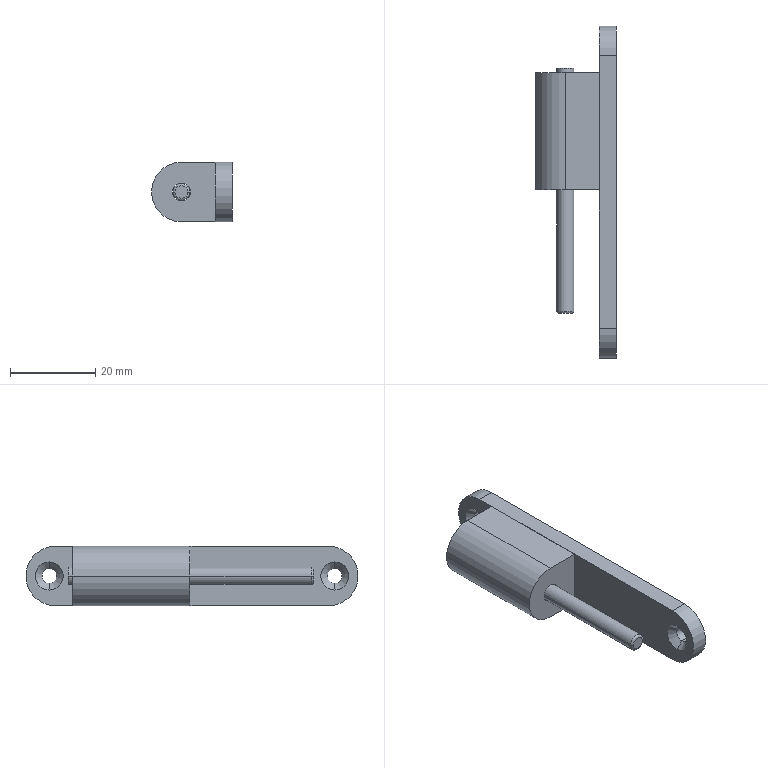Component | SolidWorks | MGL-PACK-03-00Fixture-1_MGL-PACK-03-07Hinge-1_MGL-PACK-03-07-01HingePart1-1 | 3 solids | 29 faces | box 19 x 78 x 14 mm | volume 9629 mm3 | cylinder 12 | plane 11 | cone 4 | torus 2 | commonest cylinder face diameters 14 x4 3.4 x4 4 x2 4.2 x2
build123d program:
from build123d import *

# Parameters (mm, degrees)
BOSS_EXTRUDE1_DEPTH                          = 4
BOSS_EXTRUDE2_DEPTH                          = 27.5
SKETCH5_R                                    = 2.1
CUT_EXTRUDE1_DEPTH                           = 27.5
SKETCH6_R                                    = 2
BOSS_EXTRUDE3_DEPTH                          = 57.5
FILLET1_R                                    = 0.5
HOLE_SIZE_ACCORDING_TO_PHILLIPS_COUN_2_COUNT = 2
HOLE_SIZE_ACCORDING_TO_PHILLIPS_COUN_2_PITCH = 67


with BuildPart() as part:
    # Sketch1 → Boss-Extrude1 (new body)
    with BuildSketch(Plane.XY):
        with BuildLine():
            Line((-7, 32), (-7, -32))
            ThreePointArc((-7, -32), (0, -39), (7, -32))
            Line((7, -32), (7, 32))
            ThreePointArc((7, 32), (0, 39), (-7, 32))
        make_face()
    extrude(amount=BOSS_EXTRUDE1_DEPTH)

    # Sketch7 → Hole Size according to Phillips counters (revolve, cut)
    with BuildSketch(Plane(origin=(0, 33.5, 4), x_dir=(0, -1, 0), z_dir=(1, 0, 0))):
        Polygon((0, 0), (0, 4), (1.7, 4), (1.7, 1.6), (3.3, 0), align=None)
    hole_size_according_to_phillips_counters = revolve(axis=Axis((0, 33.5, 10.35), (0, 0, -1)), mode=Mode.SUBTRACT)

    # Hole Size according to Phillips coun 2: Hole Size according to Phillips counters ×2
    with Locations(*[(0, -i * HOLE_SIZE_ACCORDING_TO_PHILLIPS_COUN_2_PITCH, 0) for i in range(1, HOLE_SIZE_ACCORDING_TO_PHILLIPS_COUN_2_COUNT)]):
        add(hole_size_according_to_phillips_counters, mode=Mode.SUBTRACT)


with BuildPart() as body_2:
    # Sketch2 → Boss-Extrude2 (new body)
    with BuildSketch(Plane(origin=(0, 28, 0), x_dir=(1, 0, 0), z_dir=(0, 1, 0))):
        with BuildLine():
            Line((-7, -4), (7, -4))
            Line((7, -4), (7, -12))
            ThreePointArc((7, -12), (0, -19), (-7, -12))
            Line((-7, -12), (-7, -4))
        make_face()
    extrude(amount=-BOSS_EXTRUDE2_DEPTH)

    # Sketch5 → Cut-Extrude1 (cut)
    with BuildSketch(Plane(origin=(0, 28, 0), x_dir=(1, 0, 0), z_dir=(0, 1, 0))):
        with Locations(Location((0, -12, 0), (0, 0, 270))):
            Circle(SKETCH5_R)
    extrude(amount=-CUT_EXTRUDE1_DEPTH, mode=Mode.SUBTRACT)


with BuildPart() as body_3:
    # Sketch6 → Boss-Extrude3 (new body)
    with BuildSketch(Plane(origin=(0, 29, 0), x_dir=(1, 0, 0), z_dir=(0, 1, 0))):
        with Locations(Location((0, -12, 0), (0, 0, 270))):
            Circle(SKETCH6_R)
    extrude(amount=-BOSS_EXTRUDE3_DEPTH)

    # Fillet1
    fillet1_edges = [body_3.edges().sort_by_distance(p)[0] for p in [
        (0, -28.5, 10),
    ]]
    fillet(fillet1_edges, radius=FILLET1_R)


solid = Compound([part.part, body_2.part, body_3.part])

# Placed as in the assembly
solid = solid.moved(Location((279.5, 0, 1.7), (0, -90, 0)))
STEP:
#1=COLOUR_RGB('',0.7922,0.8196,0.9333);
#2=FILL_AREA_STYLE_COLOUR('',#1);
#3=FILL_AREA_STYLE('',(#2));
#4=SURFACE_STYLE_FILL_AREA(#3);
#5=SURFACE_SIDE_STYLE('',(#4));
#6=SURFACE_STYLE_USAGE(.BOTH.,#5);
#7=PRESENTATION_STYLE_ASSIGNMENT((#6));
#8=CARTESIAN_POINT('',(10.909,1.319,0.));
#9=VERTEX_POINT('',#8);
#10=CARTESIAN_POINT('',(10.909,1.319,0.1339));
#11=VERTEX_POINT('',#10);
#12=CARTESIAN_POINT('',(10.909,1.319,0.06693));
#13=DIRECTION('',(-1.,-0.,0.));
#14=DIRECTION('',(0.,0.,1.));
#15=AXIS2_PLACEMENT_3D('',#12,#13,#14);
#16=CIRCLE('',#15,0.06693);
#17=EDGE_CURVE('',#9,#11,#16,.T.);
#18=ORIENTED_EDGE('',*,*,#17,.F.);
#19=CARTESIAN_POINT('',(10.846,1.319,-0.06299));
#20=VERTEX_POINT('',#19);
#21=CARTESIAN_POINT('',(10.846,1.319,-0.06299));
#22=DIRECTION('',(-0.7071,-0.,-0.7071));
#23=VECTOR('',#22,39.37);
#24=LINE('',#21,#23);
#25=EDGE_CURVE('',#9,#20,#24,.T.);
#26=ORIENTED_EDGE('',*,*,#25,.T.);
#27=CARTESIAN_POINT('',(10.846,1.319,0.1969));
#28=VERTEX_POINT('',#27);
#29=CARTESIAN_POINT('',(10.846,1.319,0.06693));
#30=DIRECTION('',(-1.,-0.,0.));
#31=DIRECTION('',(0.,0.,1.));
#32=AXIS2_PLACEMENT_3D('',#29,#30,#31);
#33=CIRCLE('',#32,0.1299);
#34=EDGE_CURVE('',#20,#28,#33,.T.);
#35=ORIENTED_EDGE('',*,*,#34,.T.);
#36=CARTESIAN_POINT('',(10.846,1.319,0.1969));
#37=DIRECTION('',(-0.7071,-0.,0.7071));
#38=VECTOR('',#37,39.37);
#39=LINE('',#36,#38);
#40=EDGE_CURVE('',#11,#28,#39,.T.);
#41=ORIENTED_EDGE('',*,*,#40,.F.);
#42=EDGE_LOOP('',(#18,#26,#35,#41));
#43=FACE_OUTER_BOUND('',#42,.T.);
#44=CARTESIAN_POINT('',(10.846,1.319,0.06693));
#45=DIRECTION('',(-1.,-0.,0.));
#46=DIRECTION('',(0.,0.,1.));
#47=AXIS2_PLACEMENT_3D('',#44,#45,#46);
#48=CONICAL_SURFACE('',#47,0.1299,0.7854);
#49=ADVANCED_FACE('',(#43),#48,.F.);
#50=CARTESIAN_POINT('',(11.004,1.319,0.));
#51=VERTEX_POINT('',#50);
#52=CARTESIAN_POINT('',(11.004,1.319,0.1339));
#53=VERTEX_POINT('',#52);
#54=CARTESIAN_POINT('',(11.004,1.319,0.06693));
#55=DIRECTION('',(-1.,-0.,0.));
#56=DIRECTION('',(0.,0.,1.));
#57=AXIS2_PLACEMENT_3D('',#54,#55,#56);
#58=CIRCLE('',#57,0.06693);
#59=EDGE_CURVE('',#51,#53,#58,.T.);
#60=ORIENTED_EDGE('',*,*,#59,.F.);
#61=CARTESIAN_POINT('',(10.846,1.319,0.));
#62=DIRECTION('',(-1.,-0.,0.));
#63=VECTOR('',#62,39.37);
#64=LINE('',#61,#63);
#65=EDGE_CURVE('',#51,#9,#64,.T.);
#66=ORIENTED_EDGE('',*,*,#65,.T.);
#67=ORIENTED_EDGE('',*,*,#17,.T.);
#68=CARTESIAN_POINT('',(10.846,1.319,0.1339));
#69=DIRECTION('',(-1.,-0.,0.));
#70=VECTOR('',#69,39.37);
#71=LINE('',#68,#70);
#72=EDGE_CURVE('',#53,#11,#71,.T.);
#73=ORIENTED_EDGE('',*,*,#72,.F.);
#74=EDGE_LOOP('',(#60,#66,#67,#73));
#75=FACE_OUTER_BOUND('',#74,.T.);
#76=CARTESIAN_POINT('',(10.846,1.319,0.06693));
#77=DIRECTION('',(-1.,-0.,0.));
#78=DIRECTION('',(0.,0.,1.));
#79=AXIS2_PLACEMENT_3D('',#76,#77,#78);
#80=CYLINDRICAL_SURFACE('',#79,0.06693);
#81=ADVANCED_FACE('',(#75),#80,.F.);
#82=CARTESIAN_POINT('',(10.909,-1.319,0.));
#83=VERTEX_POINT('',#82);
#84=CARTESIAN_POINT('',(10.909,-1.319,0.1339));
#85=VERTEX_POINT('',#84);
#86=CARTESIAN_POINT('',(10.909,-1.319,0.06693));
#87=DIRECTION('',(-1.,-0.,0.));
#88=DIRECTION('',(0.,0.,1.));
#89=AXIS2_PLACEMENT_3D('',#86,#87,#88);
#90=CIRCLE('',#89,0.06693);
#91=EDGE_CURVE('',#83,#85,#90,.T.);
#92=ORIENTED_EDGE('',*,*,#91,.F.);
#93=CARTESIAN_POINT('',(10.846,-1.319,-0.06299));
#94=VERTEX_POINT('',#93);
#95=CARTESIAN_POINT('',(10.846,-1.319,-0.06299));
#96=DIRECTION('',(-0.7071,-0.,-0.7071));
#97=VECTOR('',#96,39.37);
#98=LINE('',#95,#97);
#99=EDGE_CURVE('',#83,#94,#98,.T.);
#100=ORIENTED_EDGE('',*,*,#99,.T.);
#101=CARTESIAN_POINT('',(10.846,-1.319,0.1969));
#102=VERTEX_POINT('',#101);
#103=CARTESIAN_POINT('',(10.846,-1.319,0.06693));
#104=DIRECTION('',(-1.,-0.,0.));
#105=DIRECTION('',(0.,0.,1.));
#106=AXIS2_PLACEMENT_3D('',#103,#104,#105);
#107=CIRCLE('',#106,0.1299);
#108=EDGE_CURVE('',#94,#102,#107,.T.);
#109=ORIENTED_EDGE('',*,*,#108,.T.);
#110=CARTESIAN_POINT('',(10.846,-1.319,0.1969));
#111=DIRECTION('',(-0.7071,-0.,0.7071));
#112=VECTOR('',#111,39.37);
#113=LINE('',#110,#112);
#114=EDGE_CURVE('',#85,#102,#113,.T.);
#115=ORIENTED_EDGE('',*,*,#114,.F.);
#116=EDGE_LOOP('',(#92,#100,#109,#115));
#117=FACE_OUTER_BOUND('',#116,.T.);
#118=CARTESIAN_POINT('',(10.846,-1.319,0.06693));
#119=DIRECTION('',(-1.,-0.,0.));
#120=DIRECTION('',(0.,0.,1.));
#121=AXIS2_PLACEMENT_3D('',#118,#119,#120);
#122=CONICAL_SURFACE('',#121,0.1299,0.7854);
#123=ADVANCED_FACE('',(#117),#122,.F.);
#124=CARTESIAN_POINT('',(11.004,-1.319,0.));
#125=VERTEX_POINT('',#124);
#126=CARTESIAN_POINT('',(11.004,-1.319,0.1339));
#127=VERTEX_POINT('',#126);
#128=CARTESIAN_POINT('',(11.004,-1.319,0.06693));
#129=DIRECTION('',(-1.,-0.,0.));
#130=DIRECTION('',(0.,0.,1.));
#131=AXIS2_PLACEMENT_3D('',#128,#129,#130);
#132=CIRCLE('',#131,0.06693);
#133=EDGE_CURVE('',#125,#127,#132,.T.);
#134=ORIENTED_EDGE('',*,*,#133,.F.);
#135=CARTESIAN_POINT('',(10.846,-1.319,0.));
#136=DIRECTION('',(-1.,-0.,0.));
#137=VECTOR('',#136,39.37);
#138=LINE('',#135,#137);
#139=EDGE_CURVE('',#125,#83,#138,.T.);
#140=ORIENTED_EDGE('',*,*,#139,.T.);
#141=ORIENTED_EDGE('',*,*,#91,.T.);
#142=CARTESIAN_POINT('',(10.846,-1.319,0.1339));
#143=DIRECTION('',(-1.,-0.,0.));
#144=VECTOR('',#143,39.37);
#145=LINE('',#142,#144);
#146=EDGE_CURVE('',#127,#85,#145,.T.);
#147=ORIENTED_EDGE('',*,*,#146,.F.);
#148=EDGE_LOOP('',(#134,#140,#141,#147));
#149=FACE_OUTER_BOUND('',#148,.T.);
#150=CARTESIAN_POINT('',(10.846,-1.319,0.06693));
#151=DIRECTION('',(-1.,-0.,0.));
#152=DIRECTION('',(0.,0.,1.));
#153=AXIS2_PLACEMENT_3D('',#150,#151,#152);
#154=CYLINDRICAL_SURFACE('',#153,0.06693);
#155=ADVANCED_FACE('',(#149),#154,.F.);
#156=CARTESIAN_POINT('',(11.004,1.26,0.3425));
#157=VERTEX_POINT('',#156);
#158=CARTESIAN_POINT('',(11.004,1.26,-0.2087));
#159=VERTEX_POINT('',#158);
#160=CARTESIAN_POINT('',(11.004,1.26,0.06693));
#161=DIRECTION('',(-1.,-0.,0.));
#162=DIRECTION('',(0.,0.,1.));
#163=AXIS2_PLACEMENT_3D('',#160,#161,#162);
#164=CIRCLE('',#163,0.2756);
#165=EDGE_CURVE('',#157,#159,#164,.T.);
#166=ORIENTED_EDGE('',*,*,#165,.T.);
#167=CARTESIAN_POINT('',(10.846,1.26,-0.2087));
#168=VERTEX_POINT('',#167);
#169=CARTESIAN_POINT('',(10.846,1.26,-0.2087));
#170=DIRECTION('',(1.,0.,-0.));
#171=VECTOR('',#170,39.37);
#172=LINE('',#169,#171);
#173=EDGE_CURVE('',#168,#159,#172,.T.);
#174=ORIENTED_EDGE('',*,*,#173,.F.);
#175=CARTESIAN_POINT('',(10.846,1.26,0.3425));
#176=VERTEX_POINT('',#175);
#177=CARTESIAN_POINT('',(10.846,1.26,0.06693));
#178=DIRECTION('',(-1.,-0.,0.));
#179=DIRECTION('',(0.,0.,1.));
#180=AXIS2_PLACEMENT_3D('',#177,#178,#179);
#181=CIRCLE('',#180,0.2756);
#182=EDGE_CURVE('',#176,#168,#181,.T.);
#183=ORIENTED_EDGE('',*,*,#182,.F.);
#184=CARTESIAN_POINT('',(10.846,1.26,0.3425));
#185=DIRECTION('',(1.,0.,-0.));
#186=VECTOR('',#185,39.37);
#187=LINE('',#184,#186);
#188=EDGE_CURVE('',#176,#157,#187,.T.);
#189=ORIENTED_EDGE('',*,*,#188,.T.);
#190=EDGE_LOOP('',(#166,#174,#183,#189));
#191=FACE_OUTER_BOUND('',#190,.T.);
#192=CARTESIAN_POINT('',(10.846,1.26,0.06693));
#193=DIRECTION('',(1.,0.,-0.));
#194=DIRECTION('',(0.,0.,-1.));
#195=AXIS2_PLACEMENT_3D('',#192,#193,#194);
#196=CYLINDRICAL_SURFACE('',#195,0.2756);
#197=ADVANCED_FACE('',(#191),#196,.T.);
#198=CARTESIAN_POINT('',(11.004,-1.26,-0.2087));
#199=VERTEX_POINT('',#198);
#200=CARTESIAN_POINT('',(11.004,1.26,-0.2087));
#201=DIRECTION('',(0.,-1.,0.));
#202=VECTOR('',#201,39.37);
#203=LINE('',#200,#202);
#204=EDGE_CURVE('',#159,#199,#203,.T.);
#205=ORIENTED_EDGE('',*,*,#204,.T.);
#206=CARTESIAN_POINT('',(10.846,-1.26,-0.2087));
#207=VERTEX_POINT('',#206);
#208=CARTESIAN_POINT('',(10.846,-1.26,-0.2087));
#209=DIRECTION('',(1.,0.,-0.));
#210=VECTOR('',#209,39.37);
#211=LINE('',#208,#210);
#212=EDGE_CURVE('',#207,#199,#211,.T.);
#213=ORIENTED_EDGE('',*,*,#212,.F.);
#214=CARTESIAN_POINT('',(10.846,1.26,-0.2087));
#215=DIRECTION('',(0.,-1.,0.));
#216=VECTOR('',#215,39.37);
#217=LINE('',#214,#216);
#218=EDGE_CURVE('',#168,#207,#217,.T.);
#219=ORIENTED_EDGE('',*,*,#218,.F.);
#220=ORIENTED_EDGE('',*,*,#173,.T.);
#221=EDGE_LOOP('',(#205,#213,#219,#220));
#222=FACE_OUTER_BOUND('',#221,.T.);
#223=CARTESIAN_POINT('',(10.846,1.26,-0.2087));
#224=DIRECTION('',(0.,0.,1.));
#225=DIRECTION('',(-0.,1.,-0.));
#226=AXIS2_PLACEMENT_3D('',#223,#224,#225);
#227=PLANE('',#226);
#228=ADVANCED_FACE('',(#222),#227,.F.);
#229=CARTESIAN_POINT('',(11.004,-1.26,0.3425));
#230=VERTEX_POINT('',#229);
#231=CARTESIAN_POINT('',(11.004,-1.26,0.06693));
#232=DIRECTION('',(-1.,-0.,0.));
#233=DIRECTION('',(0.,0.,1.));
#234=AXIS2_PLACEMENT_3D('',#231,#232,#233);
#235=CIRCLE('',#234,0.2756);
#236=EDGE_CURVE('',#199,#230,#235,.T.);
#237=ORIENTED_EDGE('',*,*,#236,.T.);
#238=CARTESIAN_POINT('',(10.846,-1.26,0.3425));
#239=VERTEX_POINT('',#238);
#240=CARTESIAN_POINT('',(10.846,-1.26,0.3425));
#241=DIRECTION('',(1.,0.,-0.));
#242=VECTOR('',#241,39.37);
#243=LINE('',#240,#242);
#244=EDGE_CURVE('',#239,#230,#243,.T.);
#245=ORIENTED_EDGE('',*,*,#244,.F.);
#246=CARTESIAN_POINT('',(10.846,-1.26,0.06693));
#247=DIRECTION('',(-1.,-0.,0.));
#248=DIRECTION('',(0.,0.,1.));
#249=AXIS2_PLACEMENT_3D('',#246,#247,#248);
#250=CIRCLE('',#249,0.2756);
#251=EDGE_CURVE('',#207,#239,#250,.T.);
#252=ORIENTED_EDGE('',*,*,#251,.F.);
#253=ORIENTED_EDGE('',*,*,#212,.T.);
#254=EDGE_LOOP('',(#237,#245,#252,#253));
#255=FACE_OUTER_BOUND('',#254,.T.);
#256=CARTESIAN_POINT('',(10.846,-1.26,0.06693));
#257=DIRECTION('',(1.,0.,-0.));
#258=DIRECTION('',(0.,0.,-1.));
#259=AXIS2_PLACEMENT_3D('',#256,#257,#258);
#260=CYLINDRICAL_SURFACE('',#259,0.2756);
#261=ADVANCED_FACE('',(#255),#260,.T.);
#262=CARTESIAN_POINT('',(11.004,1.26,0.3425));
#263=DIRECTION('',(-0.,1.,-0.));
#264=VECTOR('',#263,39.37);
#265=LINE('',#262,#264);
#266=EDGE_CURVE('',#230,#157,#265,.T.);
#267=ORIENTED_EDGE('',*,*,#266,.T.);
#268=ORIENTED_EDGE('',*,*,#188,.F.);
#269=CARTESIAN_POINT('',(10.846,1.26,0.3425));
#270=DIRECTION('',(-0.,1.,-0.));
#271=VECTOR('',#270,39.37);
#272=LINE('',#269,#271);
#273=EDGE_CURVE('',#239,#176,#272,.T.);
#274=ORIENTED_EDGE('',*,*,#273,.F.);
#275=ORIENTED_EDGE('',*,*,#244,.T.);
#276=EDGE_LOOP('',(#267,#268,#274,#275));
#277=FACE_OUTER_BOUND('',#276,.T.);
#278=CARTESIAN_POINT('',(10.846,1.26,0.3425));
#279=DIRECTION('',(-0.,-0.,-1.));
#280=DIRECTION('',(0.,-1.,0.));
#281=AXIS2_PLACEMENT_3D('',#278,#279,#280);
#282=PLANE('',#281);
#283=ADVANCED_FACE('',(#277),#282,.F.);
#284=CARTESIAN_POINT('',(10.846,1.319,0.06693));
#285=DIRECTION('',(-1.,-0.,0.));
#286=DIRECTION('',(0.,0.,1.));
#287=AXIS2_PLACEMENT_3D('',#284,#285,#286);
#288=CIRCLE('',#287,0.1299);
#289=EDGE_CURVE('',#28,#20,#288,.T.);
#290=ORIENTED_EDGE('',*,*,#289,.F.);
#291=ORIENTED_EDGE('',*,*,#34,.F.);
#292=EDGE_LOOP('',(#290,#291));
#293=FACE_BOUND('',#292,.T.);
#294=CARTESIAN_POINT('',(10.846,-1.319,0.06693));
#295=DIRECTION('',(-1.,-0.,0.));
#296=DIRECTION('',(0.,0.,1.));
#297=AXIS2_PLACEMENT_3D('',#294,#295,#296);
#298=CIRCLE('',#297,0.1299);
#299=EDGE_CURVE('',#102,#94,#298,.T.);
#300=ORIENTED_EDGE('',*,*,#299,.F.);
#301=ORIENTED_EDGE('',*,*,#108,.F.);
#302=EDGE_LOOP('',(#300,#301));
#303=FACE_BOUND('',#302,.T.);
#304=ORIENTED_EDGE('',*,*,#182,.T.);
#305=ORIENTED_EDGE('',*,*,#218,.T.);
#306=ORIENTED_EDGE('',*,*,#251,.T.);
#307=ORIENTED_EDGE('',*,*,#273,.T.);
#308=EDGE_LOOP('',(#304,#305,#306,#307));
#309=FACE_OUTER_BOUND('',#308,.T.);
#310=CARTESIAN_POINT('',(10.846,1.26,0.06693));
#311=DIRECTION('',(-1.,-0.,0.));
#312=DIRECTION('',(0.,-0.,1.));
#313=AXIS2_PLACEMENT_3D('',#310,#311,#312);
#314=PLANE('',#313);
#315=ADVANCED_FACE('',(#293,#303,#309),#314,.T.);
#316=CARTESIAN_POINT('',(11.004,1.319,0.06693));
#317=DIRECTION('',(-1.,-0.,0.));
#318=DIRECTION('',(0.,0.,1.));
#319=AXIS2_PLACEMENT_3D('',#316,#317,#318);
#320=CIRCLE('',#319,0.06693);
#321=EDGE_CURVE('',#53,#51,#320,.T.);
#322=ORIENTED_EDGE('',*,*,#321,.T.);
#323=ORIENTED_EDGE('',*,*,#59,.T.);
#324=EDGE_LOOP('',(#322,#323));
#325=FACE_BOUND('',#324,.T.);
#326=CARTESIAN_POINT('',(11.004,-1.319,0.06693));
#327=DIRECTION('',(-1.,-0.,0.));
#328=DIRECTION('',(0.,0.,1.));
#329=AXIS2_PLACEMENT_3D('',#326,#327,#328);
#330=CIRCLE('',#329,0.06693);
#331=EDGE_CURVE('',#127,#125,#330,.T.);
#332=ORIENTED_EDGE('',*,*,#331,.T.);
#333=ORIENTED_EDGE('',*,*,#133,.T.);
#334=EDGE_LOOP('',(#332,#333));
#335=FACE_BOUND('',#334,.T.);
#336=ORIENTED_EDGE('',*,*,#165,.F.);
#337=ORIENTED_EDGE('',*,*,#266,.F.);
#338=ORIENTED_EDGE('',*,*,#236,.F.);
#339=ORIENTED_EDGE('',*,*,#204,.F.);
#340=EDGE_LOOP('',(#336,#337,#338,#339));
#341=FACE_OUTER_BOUND('',#340,.T.);
#342=CARTESIAN_POINT('',(11.004,1.26,0.06693));
#343=DIRECTION('',(-1.,-0.,0.));
#344=DIRECTION('',(0.,-0.,1.));
#345=AXIS2_PLACEMENT_3D('',#342,#343,#344);
#346=PLANE('',#345);
#347=ADVANCED_FACE('',(#325,#335,#341),#346,.F.);
#348=ORIENTED_EDGE('',*,*,#139,.F.);
#349=ORIENTED_EDGE('',*,*,#331,.F.);
#350=ORIENTED_EDGE('',*,*,#146,.T.);
#351=CARTESIAN_POINT('',(10.909,-1.319,0.06693));
#352=DIRECTION('',(-1.,-0.,0.));
#353=DIRECTION('',(0.,0.,1.));
#354=AXIS2_PLACEMENT_3D('',#351,#352,#353);
#355=CIRCLE('',#354,0.06693);
#356=EDGE_CURVE('',#85,#83,#355,.T.);
#357=ORIENTED_EDGE('',*,*,#356,.T.);
#358=EDGE_LOOP('',(#348,#349,#350,#357));
#359=FACE_OUTER_BOUND('',#358,.T.);
#360=CARTESIAN_POINT('',(10.846,-1.319,0.06693));
#361=DIRECTION('',(-1.,-0.,0.));
#362=DIRECTION('',(0.,0.,1.));
#363=AXIS2_PLACEMENT_3D('',#360,#361,#362);
#364=CYLINDRICAL_SURFACE('',#363,0.06693);
#365=ADVANCED_FACE('',(#359),#364,.F.);
#366=ORIENTED_EDGE('',*,*,#99,.F.);
#367=ORIENTED_EDGE('',*,*,#356,.F.);
#368=ORIENTED_EDGE('',*,*,#114,.T.);
#369=ORIENTED_EDGE('',*,*,#299,.T.);
#370=EDGE_LOOP('',(#366,#367,#368,#369));
#371=FACE_OUTER_BOUND('',#370,.T.);
#372=CARTESIAN_POINT('',(10.846,-1.319,0.06693));
#373=DIRECTION('',(-1.,-0.,0.));
#374=DIRECTION('',(0.,0.,1.));
#375=AXIS2_PLACEMENT_3D('',#372,#373,#374);
#376=CONICAL_SURFACE('',#375,0.1299,0.7854);
#377=ADVANCED_FACE('',(#371),#376,.F.);
#378=ORIENTED_EDGE('',*,*,#65,.F.);
#379=ORIENTED_EDGE('',*,*,#321,.F.);
#380=ORIENTED_EDGE('',*,*,#72,.T.);
#381=CARTESIAN_POINT('',(10.909,1.319,0.06693));
#382=DIRECTION('',(-1.,-0.,0.));
#383=DIRECTION('',(0.,0.,1.));
#384=AXIS2_PLACEMENT_3D('',#381,#382,#383);
#385=CIRCLE('',#384,0.06693);
#386=EDGE_CURVE('',#11,#9,#385,.T.);
#387=ORIENTED_EDGE('',*,*,#386,.T.);
#388=EDGE_LOOP('',(#378,#379,#380,#387));
#389=FACE_OUTER_BOUND('',#388,.T.);
#390=CARTESIAN_POINT('',(10.846,1.319,0.06693));
#391=DIRECTION('',(-1.,-0.,0.));
#392=DIRECTION('',(0.,0.,1.));
#393=AXIS2_PLACEMENT_3D('',#390,#391,#392);
#394=CYLINDRICAL_SURFACE('',#393,0.06693);
#395=ADVANCED_FACE('',(#389),#394,.F.);
#396=ORIENTED_EDGE('',*,*,#25,.F.);
#397=ORIENTED_EDGE('',*,*,#386,.F.);
#398=ORIENTED_EDGE('',*,*,#40,.T.);
#399=ORIENTED_EDGE('',*,*,#289,.T.);
#400=EDGE_LOOP('',(#396,#397,#398,#399));
#401=FACE_OUTER_BOUND('',#400,.T.);
#402=CARTESIAN_POINT('',(10.846,1.319,0.06693));
#403=DIRECTION('',(-1.,-0.,0.));
#404=DIRECTION('',(0.,0.,1.));
#405=AXIS2_PLACEMENT_3D('',#402,#403,#404);
#406=CONICAL_SURFACE('',#405,0.1299,0.7854);
#407=ADVANCED_FACE('',(#401),#406,.F.);
#408=CLOSED_SHELL('',(#49,#81,#123,#155,#197,#228,#261,#283,#315,#347,#365,#377,#395,#407));
#409=MANIFOLD_SOLID_BREP('',#408);
#410=STYLED_ITEM('',(#7),#409);
#411=PRESENTATION_LAYER_ASSIGNMENT('','',(#410));
#412=(LENGTH_UNIT()NAMED_UNIT(*)SI_UNIT($,.METRE.));
#413=LENGTH_MEASURE_WITH_UNIT(LENGTH_MEASURE(0.0254),#412);
#414=DIMENSIONAL_EXPONENTS(1.,0.,0.,0.,0.,0.,0.);
#415=(CONVERSION_BASED_UNIT('',#413)LENGTH_UNIT()NAMED_UNIT(#414));
#416=UNCERTAINTY_MEASURE_WITH_UNIT(LENGTH_MEASURE(0.00001),#415,'','');
#417=(NAMED_UNIT(*)PLANE_ANGLE_UNIT()SI_UNIT($,.RADIAN.));
#418=(NAMED_UNIT(*)SI_UNIT($,.STERADIAN.)SOLID_ANGLE_UNIT());
#419=(GEOMETRIC_REPRESENTATION_CONTEXT(3)GLOBAL_UNCERTAINTY_ASSIGNED_CONTEXT((#416))GLOBAL_UNIT_ASSIGNED_CONTEXT((#415,#417,#418))REPRESENTATION_CONTEXT('',''));
#420=MECHANICAL_DESIGN_GEOMETRIC_PRESENTATION_REPRESENTATION('',(#410),#419);
#421=COLOUR_RGB('',0.7922,0.8196,0.9333);
#422=FILL_AREA_STYLE_COLOUR('',#421);
#423=FILL_AREA_STYLE('',(#422));
#424=SURFACE_STYLE_FILL_AREA(#423);
#425=SURFACE_SIDE_STYLE('',(#424));
#426=SURFACE_STYLE_USAGE(.BOTH.,#425);
#427=PRESENTATION_STYLE_ASSIGNMENT((#426));
#428=CARTESIAN_POINT('',(10.591,-1.122,0.06693));
#429=VERTEX_POINT('',#428);
#430=CARTESIAN_POINT('',(10.472,-1.122,0.06693));
#431=VERTEX_POINT('',#430);
#432=CARTESIAN_POINT('',(10.531,-1.122,0.06693));
#433=DIRECTION('',(0.,-1.,-0.));
#434=DIRECTION('',(-1.,0.,0.));
#435=AXIS2_PLACEMENT_3D('',#432,#433,#434);
#436=CIRCLE('',#435,0.05906);
#437=EDGE_CURVE('',#429,#431,#436,.T.);
#438=ORIENTED_EDGE('',*,*,#437,.F.);
#439=CARTESIAN_POINT('',(10.61,-1.102,0.06693));
#440=VERTEX_POINT('',#439);
#441=CARTESIAN_POINT('',(10.591,-1.102,0.06693));
#442=DIRECTION('',(0.,-0.,1.));
#443=DIRECTION('',(0.,-1.,0.));
#444=AXIS2_PLACEMENT_3D('',#441,#442,#443);
#445=CIRCLE('',#444,0.01969);
#446=EDGE_CURVE('',#429,#440,#445,.T.);
#447=ORIENTED_EDGE('',*,*,#446,.T.);
#448=CARTESIAN_POINT('',(10.453,-1.102,0.06693));
#449=VERTEX_POINT('',#448);
#450=CARTESIAN_POINT('',(10.531,-1.102,0.06693));
#451=DIRECTION('',(-0.,1.,0.));
#452=DIRECTION('',(-1.,0.,0.));
#453=AXIS2_PLACEMENT_3D('',#450,#451,#452);
#454=CIRCLE('',#453,0.07874);
#455=EDGE_CURVE('',#449,#440,#454,.T.);
#456=ORIENTED_EDGE('',*,*,#455,.F.);
#457=CARTESIAN_POINT('',(10.472,-1.102,0.06693));
#458=DIRECTION('',(-0.,0.,-1.));
#459=DIRECTION('',(-1.,0.,0.));
#460=AXIS2_PLACEMENT_3D('',#457,#458,#459);
#461=CIRCLE('',#460,0.01969);
#462=EDGE_CURVE('',#431,#449,#461,.T.);
#463=ORIENTED_EDGE('',*,*,#462,.F.);
#464=EDGE_LOOP('',(#438,#447,#456,#463));
#465=FACE_OUTER_BOUND('',#464,.T.);
#466=CARTESIAN_POINT('',(10.531,-1.102,0.06693));
#467=DIRECTION('',(-0.,1.,0.));
#468=DIRECTION('',(-1.,-0.,0.));
#469=AXIS2_PLACEMENT_3D('',#466,#467,#468);
#470=TOROIDAL_SURFACE('',#469,0.05906,0.01969);
#471=ADVANCED_FACE('',(#465),#470,.T.);
#472=ORIENTED_EDGE('',*,*,#455,.T.);
#473=CARTESIAN_POINT('',(10.61,1.142,0.06693));
#474=VERTEX_POINT('',#473);
#475=CARTESIAN_POINT('',(10.61,-1.122,0.06693));
#476=DIRECTION('',(-0.,1.,0.));
#477=VECTOR('',#476,39.37);
#478=LINE('',#475,#477);
#479=EDGE_CURVE('',#440,#474,#478,.T.);
#480=ORIENTED_EDGE('',*,*,#479,.T.);
#481=CARTESIAN_POINT('',(10.453,1.142,0.06693));
#482=VERTEX_POINT('',#481);
#483=CARTESIAN_POINT('',(10.531,1.142,0.06693));
#484=DIRECTION('',(-0.,1.,0.));
#485=DIRECTION('',(-1.,0.,0.));
#486=AXIS2_PLACEMENT_3D('',#483,#484,#485);
#487=CIRCLE('',#486,0.07874);
#488=EDGE_CURVE('',#482,#474,#487,.T.);
#489=ORIENTED_EDGE('',*,*,#488,.F.);
#490=CARTESIAN_POINT('',(10.453,-1.122,0.06693));
#491=DIRECTION('',(-0.,1.,0.));
#492=VECTOR('',#491,39.37);
#493=LINE('',#490,#492);
#494=EDGE_CURVE('',#449,#482,#493,.T.);
#495=ORIENTED_EDGE('',*,*,#494,.F.);
#496=EDGE_LOOP('',(#472,#480,#489,#495));
#497=FACE_OUTER_BOUND('',#496,.T.);
#498=CARTESIAN_POINT('',(10.531,-1.122,0.06693));
#499=DIRECTION('',(-0.,1.,0.));
#500=DIRECTION('',(-1.,0.,0.));
#501=AXIS2_PLACEMENT_3D('',#498,#499,#500);
#502=CYLINDRICAL_SURFACE('',#501,0.07874);
#503=ADVANCED_FACE('',(#497),#502,.T.);
#504=ORIENTED_EDGE('',*,*,#479,.F.);
#505=CARTESIAN_POINT('',(10.531,-1.102,0.06693));
#506=DIRECTION('',(-0.,1.,0.));
#507=DIRECTION('',(-1.,0.,0.));
#508=AXIS2_PLACEMENT_3D('',#505,#506,#507);
#509=CIRCLE('',#508,0.07874);
#510=EDGE_CURVE('',#440,#449,#509,.T.);
#511=ORIENTED_EDGE('',*,*,#510,.T.);
#512=ORIENTED_EDGE('',*,*,#494,.T.);
#513=CARTESIAN_POINT('',(10.531,1.142,0.06693));
#514=DIRECTION('',(-0.,1.,0.));
#515=DIRECTION('',(-1.,0.,0.));
#516=AXIS2_PLACEMENT_3D('',#513,#514,#515);
#517=CIRCLE('',#516,0.07874);
#518=EDGE_CURVE('',#474,#482,#517,.T.);
#519=ORIENTED_EDGE('',*,*,#518,.F.);
#520=EDGE_LOOP('',(#504,#511,#512,#519));
#521=FACE_OUTER_BOUND('',#520,.T.);
#522=CARTESIAN_POINT('',(10.531,-1.122,0.06693));
#523=DIRECTION('',(-0.,1.,0.));
#524=DIRECTION('',(-1.,0.,0.));
#525=AXIS2_PLACEMENT_3D('',#522,#523,#524);
#526=CYLINDRICAL_SURFACE('',#525,0.07874);
#527=ADVANCED_FACE('',(#521),#526,.T.);
#528=CARTESIAN_POINT('',(10.531,-1.122,0.06693));
#529=DIRECTION('',(0.,-1.,-0.));
#530=DIRECTION('',(-1.,0.,0.));
#531=AXIS2_PLACEMENT_3D('',#528,#529,#530);
#532=CIRCLE('',#531,0.05906);
#533=EDGE_CURVE('',#431,#429,#532,.T.);
#534=ORIENTED_EDGE('',*,*,#533,.T.);
#535=ORIENTED_EDGE('',*,*,#437,.T.);
#536=EDGE_LOOP('',(#534,#535));
#537=FACE_OUTER_BOUND('',#536,.T.);
#538=CARTESIAN_POINT('',(10.531,-1.122,0.06693));
#539=DIRECTION('',(-0.,1.,0.));
#540=DIRECTION('',(-1.,-0.,0.));
#541=AXIS2_PLACEMENT_3D('',#538,#539,#540);
#542=PLANE('',#541);
#543=ADVANCED_FACE('',(#537),#542,.F.);
#544=ORIENTED_EDGE('',*,*,#488,.T.);
#545=ORIENTED_EDGE('',*,*,#518,.T.);
#546=EDGE_LOOP('',(#544,#545));
#547=FACE_OUTER_BOUND('',#546,.T.);
#548=CARTESIAN_POINT('',(10.531,1.142,0.06693));
#549=DIRECTION('',(-0.,1.,0.));
#550=DIRECTION('',(-1.,-0.,0.));
#551=AXIS2_PLACEMENT_3D('',#548,#549,#550);
#552=PLANE('',#551);
#553=ADVANCED_FACE('',(#547),#552,.T.);
#554=ORIENTED_EDGE('',*,*,#446,.F.);
#555=ORIENTED_EDGE('',*,*,#533,.F.);
#556=ORIENTED_EDGE('',*,*,#462,.T.);
#557=ORIENTED_EDGE('',*,*,#510,.F.);
#558=EDGE_LOOP('',(#554,#555,#556,#557));
#559=FACE_OUTER_BOUND('',#558,.T.);
#560=CARTESIAN_POINT('',(10.531,-1.102,0.06693));
#561=DIRECTION('',(-0.,1.,0.));
#562=DIRECTION('',(-1.,-0.,0.));
#563=AXIS2_PLACEMENT_3D('',#560,#561,#562);
#564=TOROIDAL_SURFACE('',#563,0.05906,0.01969);
#565=ADVANCED_FACE('',(#559),#564,.T.);
#566=CLOSED_SHELL('',(#471,#503,#527,#543,#553,#565));
#567=MANIFOLD_SOLID_BREP('',#566);
#568=STYLED_ITEM('',(#427),#567);
#569=(LENGTH_UNIT()NAMED_UNIT(*)SI_UNIT($,.METRE.));
#570=LENGTH_MEASURE_WITH_UNIT(LENGTH_MEASURE(0.0254),#569);
#571=DIMENSIONAL_EXPONENTS(1.,0.,0.,0.,0.,0.,0.);
#572=(CONVERSION_BASED_UNIT('',#570)LENGTH_UNIT()NAMED_UNIT(#571));
#573=UNCERTAINTY_MEASURE_WITH_UNIT(LENGTH_MEASURE(0.00001),#572,'','');
#574=(NAMED_UNIT(*)PLANE_ANGLE_UNIT()SI_UNIT($,.RADIAN.));
#575=(NAMED_UNIT(*)SI_UNIT($,.STERADIAN.)SOLID_ANGLE_UNIT());
#576=(GEOMETRIC_REPRESENTATION_CONTEXT(3)GLOBAL_UNCERTAINTY_ASSIGNED_CONTEXT((#573))GLOBAL_UNIT_ASSIGNED_CONTEXT((#572,#574,#575))REPRESENTATION_CONTEXT('',''));
#577=MECHANICAL_DESIGN_GEOMETRIC_PRESENTATION_REPRESENTATION('',(#568),#576);
#578=CARTESIAN_POINT('',(10.614,0.01969,0.06693));
#579=VERTEX_POINT('',#578);
#580=CARTESIAN_POINT('',(10.449,0.01969,0.06693));
#581=VERTEX_POINT('',#580);
#582=CARTESIAN_POINT('',(10.531,0.01969,0.06693));
#583=DIRECTION('',(-0.,1.,0.));
#584=DIRECTION('',(-1.,-0.,0.));
#585=AXIS2_PLACEMENT_3D('',#582,#583,#584);
#586=CIRCLE('',#585,0.08268);
#587=EDGE_CURVE('',#579,#581,#586,.T.);
#588=ORIENTED_EDGE('',*,*,#587,.F.);
#589=CARTESIAN_POINT('',(10.614,1.102,0.06693));
#590=VERTEX_POINT('',#589);
#591=CARTESIAN_POINT('',(10.614,0.01969,0.06693));
#592=DIRECTION('',(-0.,1.,0.));
#593=VECTOR('',#592,39.37);
#594=LINE('',#591,#593);
#595=EDGE_CURVE('',#579,#590,#594,.T.);
#596=ORIENTED_EDGE('',*,*,#595,.T.);
#597=CARTESIAN_POINT('',(10.449,1.102,0.06693));
#598=VERTEX_POINT('',#597);
#599=CARTESIAN_POINT('',(10.531,1.102,0.06693));
#600=DIRECTION('',(-0.,1.,0.));
#601=DIRECTION('',(-1.,0.,0.));
#602=AXIS2_PLACEMENT_3D('',#599,#600,#601);
#603=CIRCLE('',#602,0.08268);
#604=EDGE_CURVE('',#590,#598,#603,.T.);
#605=ORIENTED_EDGE('',*,*,#604,.T.);
#606=CARTESIAN_POINT('',(10.449,0.01969,0.06693));
#607=DIRECTION('',(-0.,1.,0.));
#608=VECTOR('',#607,39.37);
#609=LINE('',#606,#608);
#610=EDGE_CURVE('',#581,#598,#609,.T.);
#611=ORIENTED_EDGE('',*,*,#610,.F.);
#612=EDGE_LOOP('',(#588,#596,#605,#611));
#613=FACE_OUTER_BOUND('',#612,.T.);
#614=CARTESIAN_POINT('',(10.531,0.01969,0.06693));
#615=DIRECTION('',(-0.,1.,0.));
#616=DIRECTION('',(-1.,-0.,0.));
#617=AXIS2_PLACEMENT_3D('',#614,#615,#616);
#618=CYLINDRICAL_SURFACE('',#617,0.08268);
#619=ADVANCED_FACE('',(#613),#618,.F.);
#620=CARTESIAN_POINT('',(10.531,0.01969,-0.2087));
#621=VERTEX_POINT('',#620);
#622=CARTESIAN_POINT('',(10.256,0.01969,0.06693));
#623=VERTEX_POINT('',#622);
#624=CARTESIAN_POINT('',(10.531,0.01969,0.06693));
#625=DIRECTION('',(-0.,1.,0.));
#626=DIRECTION('',(-1.,-0.,0.));
#627=AXIS2_PLACEMENT_3D('',#624,#625,#626);
#628=CIRCLE('',#627,0.2756);
#629=EDGE_CURVE('',#621,#623,#628,.T.);
#630=ORIENTED_EDGE('',*,*,#629,.T.);
#631=CARTESIAN_POINT('',(10.256,1.102,0.06693));
#632=VERTEX_POINT('',#631);
#633=CARTESIAN_POINT('',(10.256,0.01969,0.06693));
#634=DIRECTION('',(-0.,1.,0.));
#635=VECTOR('',#634,39.37);
#636=LINE('',#633,#635);
#637=EDGE_CURVE('',#623,#632,#636,.T.);
#638=ORIENTED_EDGE('',*,*,#637,.T.);
#639=CARTESIAN_POINT('',(10.531,1.102,-0.2087));
#640=VERTEX_POINT('',#639);
#641=CARTESIAN_POINT('',(10.531,1.102,0.06693));
#642=DIRECTION('',(-0.,1.,0.));
#643=DIRECTION('',(-1.,0.,0.));
#644=AXIS2_PLACEMENT_3D('',#641,#642,#643);
#645=CIRCLE('',#644,0.2756);
#646=EDGE_CURVE('',#640,#632,#645,.T.);
#647=ORIENTED_EDGE('',*,*,#646,.F.);
#648=CARTESIAN_POINT('',(10.531,0.01969,-0.2087));
#649=DIRECTION('',(-0.,1.,0.));
#650=VECTOR('',#649,39.37);
#651=LINE('',#648,#650);
#652=EDGE_CURVE('',#621,#640,#651,.T.);
#653=ORIENTED_EDGE('',*,*,#652,.F.);
#654=EDGE_LOOP('',(#630,#638,#647,#653));
#655=FACE_OUTER_BOUND('',#654,.T.);
#656=CARTESIAN_POINT('',(10.531,0.01969,0.06693));
#657=DIRECTION('',(-0.,1.,0.));
#658=DIRECTION('',(-1.,-0.,0.));
#659=AXIS2_PLACEMENT_3D('',#656,#657,#658);
#660=CYLINDRICAL_SURFACE('',#659,0.2756);
#661=ADVANCED_FACE('',(#655),#660,.T.);
#662=CARTESIAN_POINT('',(10.846,1.102,-0.2087));
#663=VERTEX_POINT('',#662);
#664=CARTESIAN_POINT('',(10.846,1.102,-0.2087));
#665=DIRECTION('',(-1.,-0.,0.));
#666=VECTOR('',#665,39.37);
#667=LINE('',#664,#666);
#668=EDGE_CURVE('',#663,#640,#667,.T.);
#669=ORIENTED_EDGE('',*,*,#668,.F.);
#670=CARTESIAN_POINT('',(10.846,0.01969,-0.2087));
#671=VERTEX_POINT('',#670);
#672=CARTESIAN_POINT('',(10.846,0.01969,-0.2087));
#673=DIRECTION('',(-0.,1.,0.));
#674=VECTOR('',#673,39.37);
#675=LINE('',#672,#674);
#676=EDGE_CURVE('',#671,#663,#675,.T.);
#677=ORIENTED_EDGE('',*,*,#676,.F.);
#678=CARTESIAN_POINT('',(10.846,0.01969,-0.2087));
#679=DIRECTION('',(-1.,-0.,0.));
#680=VECTOR('',#679,39.37);
#681=LINE('',#678,#680);
#682=EDGE_CURVE('',#671,#621,#681,.T.);
#683=ORIENTED_EDGE('',*,*,#682,.T.);
#684=ORIENTED_EDGE('',*,*,#652,.T.);
#685=EDGE_LOOP('',(#669,#677,#683,#684));
#686=FACE_OUTER_BOUND('',#685,.T.);
#687=CARTESIAN_POINT('',(10.846,0.01969,-0.2087));
#688=DIRECTION('',(-0.,0.,-1.));
#689=DIRECTION('',(-1.,-0.,0.));
#690=AXIS2_PLACEMENT_3D('',#687,#688,#689);
#691=PLANE('',#690);
#692=ADVANCED_FACE('',(#686),#691,.T.);
#693=CARTESIAN_POINT('',(10.846,1.102,0.3425));
#694=VERTEX_POINT('',#693);
#695=CARTESIAN_POINT('',(10.846,1.102,-0.2087));
#696=DIRECTION('',(-0.,0.,-1.));
#697=VECTOR('',#696,39.37);
#698=LINE('',#695,#697);
#699=EDGE_CURVE('',#694,#663,#698,.T.);
#700=ORIENTED_EDGE('',*,*,#699,.F.);
#701=CARTESIAN_POINT('',(10.846,0.01969,0.3425));
#702=VERTEX_POINT('',#701);
#703=CARTESIAN_POINT('',(10.846,0.01969,0.3425));
#704=DIRECTION('',(-0.,1.,0.));
#705=VECTOR('',#704,39.37);
#706=LINE('',#703,#705);
#707=EDGE_CURVE('',#702,#694,#706,.T.);
#708=ORIENTED_EDGE('',*,*,#707,.F.);
#709=CARTESIAN_POINT('',(10.846,0.01969,-0.2087));
#710=DIRECTION('',(-0.,0.,-1.));
#711=VECTOR('',#710,39.37);
#712=LINE('',#709,#711);
#713=EDGE_CURVE('',#702,#671,#712,.T.);
#714=ORIENTED_EDGE('',*,*,#713,.T.);
#715=ORIENTED_EDGE('',*,*,#676,.T.);
#716=EDGE_LOOP('',(#700,#708,#714,#715));
#717=FACE_OUTER_BOUND('',#716,.T.);
#718=CARTESIAN_POINT('',(10.846,0.01969,-0.2087));
#719=DIRECTION('',(1.,0.,-0.));
#720=DIRECTION('',(-0.,0.,-1.));
#721=AXIS2_PLACEMENT_3D('',#718,#719,#720);
#722=PLANE('',#721);
#723=ADVANCED_FACE('',(#717),#722,.T.);
#724=CARTESIAN_POINT('',(10.531,1.102,0.3425));
#725=VERTEX_POINT('',#724);
#726=CARTESIAN_POINT('',(10.846,1.102,0.3425));
#727=DIRECTION('',(1.,0.,-0.));
#728=VECTOR('',#727,39.37);
#729=LINE('',#726,#728);
#730=EDGE_CURVE('',#725,#694,#729,.T.);
#731=ORIENTED_EDGE('',*,*,#730,.F.);
#732=CARTESIAN_POINT('',(10.531,0.01969,0.3425));
#733=VERTEX_POINT('',#732);
#734=CARTESIAN_POINT('',(10.531,0.01969,0.3425));
#735=DIRECTION('',(-0.,1.,0.));
#736=VECTOR('',#735,39.37);
#737=LINE('',#734,#736);
#738=EDGE_CURVE('',#733,#725,#737,.T.);
#739=ORIENTED_EDGE('',*,*,#738,.F.);
#740=CARTESIAN_POINT('',(10.846,0.01969,0.3425));
#741=DIRECTION('',(1.,0.,-0.));
#742=VECTOR('',#741,39.37);
#743=LINE('',#740,#742);
#744=EDGE_CURVE('',#733,#702,#743,.T.);
#745=ORIENTED_EDGE('',*,*,#744,.T.);
#746=ORIENTED_EDGE('',*,*,#707,.T.);
#747=EDGE_LOOP('',(#731,#739,#745,#746));
#748=FACE_OUTER_BOUND('',#747,.T.);
#749=CARTESIAN_POINT('',(10.846,0.01969,0.3425));
#750=DIRECTION('',(0.,-0.,1.));
#751=DIRECTION('',(1.,0.,-0.));
#752=AXIS2_PLACEMENT_3D('',#749,#750,#751);
#753=PLANE('',#752);
#754=ADVANCED_FACE('',(#748),#753,.T.);
#755=ORIENTED_EDGE('',*,*,#637,.F.);
#756=CARTESIAN_POINT('',(10.531,0.01969,0.06693));
#757=DIRECTION('',(-0.,1.,0.));
#758=DIRECTION('',(-1.,-0.,0.));
#759=AXIS2_PLACEMENT_3D('',#756,#757,#758);
#760=CIRCLE('',#759,0.2756);
#761=EDGE_CURVE('',#623,#733,#760,.T.);
#762=ORIENTED_EDGE('',*,*,#761,.T.);
#763=ORIENTED_EDGE('',*,*,#738,.T.);
#764=CARTESIAN_POINT('',(10.531,1.102,0.06693));
#765=DIRECTION('',(-0.,1.,0.));
#766=DIRECTION('',(-1.,0.,0.));
#767=AXIS2_PLACEMENT_3D('',#764,#765,#766);
#768=CIRCLE('',#767,0.2756);
#769=EDGE_CURVE('',#632,#725,#768,.T.);
#770=ORIENTED_EDGE('',*,*,#769,.F.);
#771=EDGE_LOOP('',(#755,#762,#763,#770));
#772=FACE_OUTER_BOUND('',#771,.T.);
#773=CARTESIAN_POINT('',(10.531,0.01969,0.06693));
#774=DIRECTION('',(-0.,1.,0.));
#775=DIRECTION('',(-1.,-0.,0.));
#776=AXIS2_PLACEMENT_3D('',#773,#774,#775);
#777=CYLINDRICAL_SURFACE('',#776,0.2756);
#778=ADVANCED_FACE('',(#772),#777,.T.);
#779=CARTESIAN_POINT('',(10.531,0.01969,0.06693));
#780=DIRECTION('',(-0.,1.,0.));
#781=DIRECTION('',(-1.,-0.,0.));
#782=AXIS2_PLACEMENT_3D('',#779,#780,#781);
#783=CIRCLE('',#782,0.08268);
#784=EDGE_CURVE('',#581,#579,#783,.T.);
#785=ORIENTED_EDGE('',*,*,#784,.T.);
#786=ORIENTED_EDGE('',*,*,#587,.T.);
#787=EDGE_LOOP('',(#785,#786));
#788=FACE_BOUND('',#787,.T.);
#789=ORIENTED_EDGE('',*,*,#682,.F.);
#790=ORIENTED_EDGE('',*,*,#713,.F.);
#791=ORIENTED_EDGE('',*,*,#744,.F.);
#792=ORIENTED_EDGE('',*,*,#761,.F.);
#793=ORIENTED_EDGE('',*,*,#629,.F.);
#794=EDGE_LOOP('',(#789,#790,#791,#792,#793));
#795=FACE_OUTER_BOUND('',#794,.T.);
#796=CARTESIAN_POINT('',(10.531,0.01969,0.06693));
#797=DIRECTION('',(-0.,1.,0.));
#798=DIRECTION('',(-1.,-0.,0.));
#799=AXIS2_PLACEMENT_3D('',#796,#797,#798);
#800=PLANE('',#799);
#801=ADVANCED_FACE('',(#788,#795),#800,.F.);
#802=CARTESIAN_POINT('',(10.531,1.102,0.06693));
#803=DIRECTION('',(-0.,1.,0.));
#804=DIRECTION('',(-1.,0.,0.));
#805=AXIS2_PLACEMENT_3D('',#802,#803,#804);
#806=CIRCLE('',#805,0.08268);
#807=EDGE_CURVE('',#598,#590,#806,.T.);
#808=ORIENTED_EDGE('',*,*,#807,.F.);
#809=ORIENTED_EDGE('',*,*,#604,.F.);
#810=EDGE_LOOP('',(#808,#809));
#811=FACE_BOUND('',#810,.T.);
#812=ORIENTED_EDGE('',*,*,#668,.T.);
#813=ORIENTED_EDGE('',*,*,#646,.T.);
#814=ORIENTED_EDGE('',*,*,#769,.T.);
#815=ORIENTED_EDGE('',*,*,#730,.T.);
#816=ORIENTED_EDGE('',*,*,#699,.T.);
#817=EDGE_LOOP('',(#812,#813,#814,#815,#816));
#818=FACE_OUTER_BOUND('',#817,.T.);
#819=CARTESIAN_POINT('',(10.531,1.102,0.06693));
#820=DIRECTION('',(-0.,1.,0.));
#821=DIRECTION('',(-1.,-0.,0.));
#822=AXIS2_PLACEMENT_3D('',#819,#820,#821);
#823=PLANE('',#822);
#824=ADVANCED_FACE('',(#811,#818),#823,.T.);
#825=ORIENTED_EDGE('',*,*,#595,.F.);
#826=ORIENTED_EDGE('',*,*,#784,.F.);
#827=ORIENTED_EDGE('',*,*,#610,.T.);
#828=ORIENTED_EDGE('',*,*,#807,.T.);
#829=EDGE_LOOP('',(#825,#826,#827,#828));
#830=FACE_OUTER_BOUND('',#829,.T.);
#831=CARTESIAN_POINT('',(10.531,0.01969,0.06693));
#832=DIRECTION('',(-0.,1.,0.));
#833=DIRECTION('',(-1.,-0.,0.));
#834=AXIS2_PLACEMENT_3D('',#831,#832,#833);
#835=CYLINDRICAL_SURFACE('',#834,0.08268);
#836=ADVANCED_FACE('',(#830),#835,.F.);
#837=CLOSED_SHELL('',(#619,#661,#692,#723,#754,#778,#801,#824,#836));
#838=MANIFOLD_SOLID_BREP('',#837);
#839=CARTESIAN_POINT('',(0.,0.,0.));
#840=DIRECTION('',(0.,0.,1.));
#841=DIRECTION('',(1.,0.,0.));
#842=AXIS2_PLACEMENT_3D('',#839,#840,#841);
#843=(LENGTH_UNIT()NAMED_UNIT(*)SI_UNIT($,.METRE.));
#844=LENGTH_MEASURE_WITH_UNIT(LENGTH_MEASURE(0.0254),#843);
#845=DIMENSIONAL_EXPONENTS(1.,0.,0.,0.,0.,0.,0.);
#846=(CONVERSION_BASED_UNIT('',#844)LENGTH_UNIT()NAMED_UNIT(#845));
#847=UNCERTAINTY_MEASURE_WITH_UNIT(LENGTH_MEASURE(0.00001),#846,'','');
#848=(NAMED_UNIT(*)PLANE_ANGLE_UNIT()SI_UNIT($,.RADIAN.));
#849=(NAMED_UNIT(*)SI_UNIT($,.STERADIAN.)SOLID_ANGLE_UNIT());
#850=(GEOMETRIC_REPRESENTATION_CONTEXT(3)GLOBAL_UNCERTAINTY_ASSIGNED_CONTEXT((#847))GLOBAL_UNIT_ASSIGNED_CONTEXT((#846,#848,#849))REPRESENTATION_CONTEXT('',''));
#851=ADVANCED_BREP_SHAPE_REPRESENTATION('',(#567,#838,#409,#842),#850);
#852=COLOUR_RGB('',0.7922,0.8196,0.9333);
#853=FILL_AREA_STYLE_COLOUR('',#852);
#854=FILL_AREA_STYLE('',(#853));
#855=SURFACE_STYLE_FILL_AREA(#854);
#856=SURFACE_SIDE_STYLE('',(#855));
#857=SURFACE_STYLE_USAGE(.BOTH.,#856);
#858=PRESENTATION_STYLE_ASSIGNMENT((#857));
#859=STYLED_ITEM('',(#858),#838);
#860=(LENGTH_UNIT()NAMED_UNIT(*)SI_UNIT($,.METRE.));
#861=LENGTH_MEASURE_WITH_UNIT(LENGTH_MEASURE(0.0254),#860);
#862=DIMENSIONAL_EXPONENTS(1.,0.,0.,0.,0.,0.,0.);
#863=(CONVERSION_BASED_UNIT('',#861)LENGTH_UNIT()NAMED_UNIT(#862));
#864=UNCERTAINTY_MEASURE_WITH_UNIT(LENGTH_MEASURE(0.00001),#863,'','');
#865=(NAMED_UNIT(*)PLANE_ANGLE_UNIT()SI_UNIT($,.RADIAN.));
#866=(NAMED_UNIT(*)SI_UNIT($,.STERADIAN.)SOLID_ANGLE_UNIT());
#867=(GEOMETRIC_REPRESENTATION_CONTEXT(3)GLOBAL_UNCERTAINTY_ASSIGNED_CONTEXT((#864))GLOBAL_UNIT_ASSIGNED_CONTEXT((#863,#865,#866))REPRESENTATION_CONTEXT('',''));
#868=MECHANICAL_DESIGN_GEOMETRIC_PRESENTATION_REPRESENTATION('',(#859),#867);
#869=PRESENTATION_LAYER_ASSIGNMENT('','',(#568));
#870=PRESENTATION_LAYER_ASSIGNMENT('','',(#859));